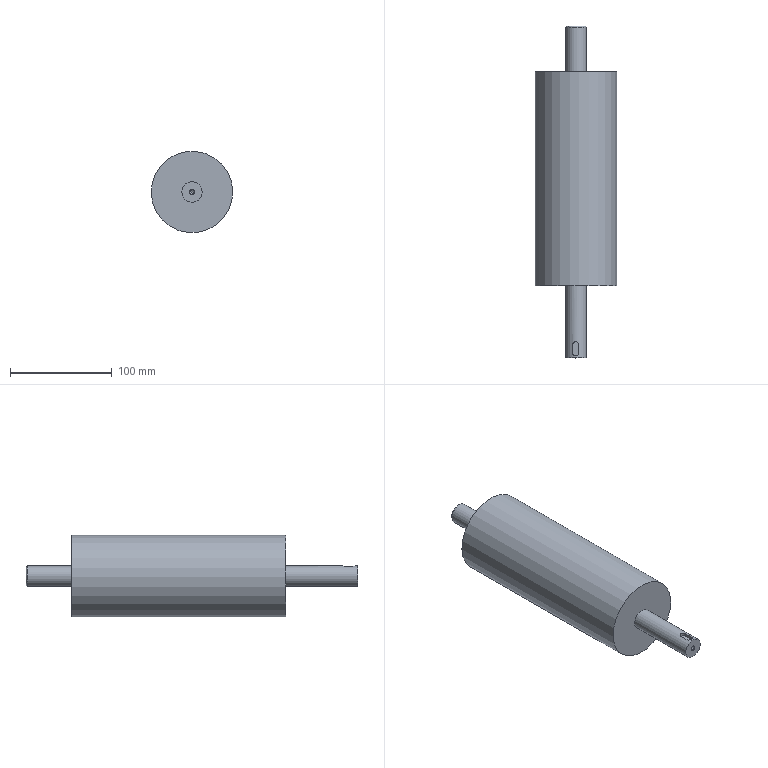Component | NX | 131_DRIVE_END_ROLLER | 1 solid | 16 faces | volume 1091585 mm3 | plane 7 | cylinder 6 | cone 3 | commonest cylinder face diameters 20 x2 6 x2 4.2 x1 80 x1